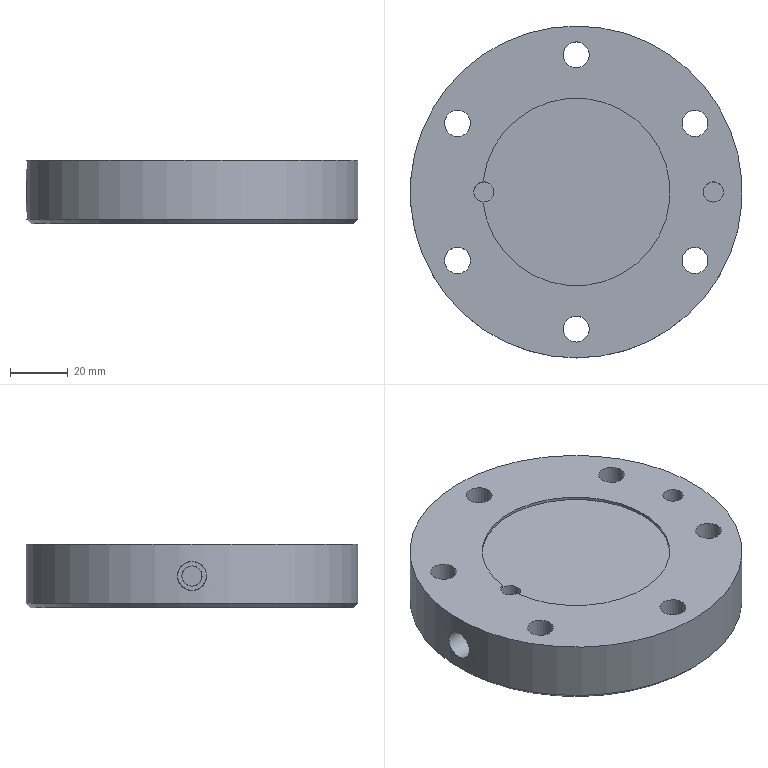Component | NX | REAR_COVER | 1 solid | 37 faces | volume 205122 mm3 | cylinder 23 | plane 13 | cone 1 | commonest cylinder face diameters 7 x8 9 x6 14 x6 115 x1 65 x1 10 x1